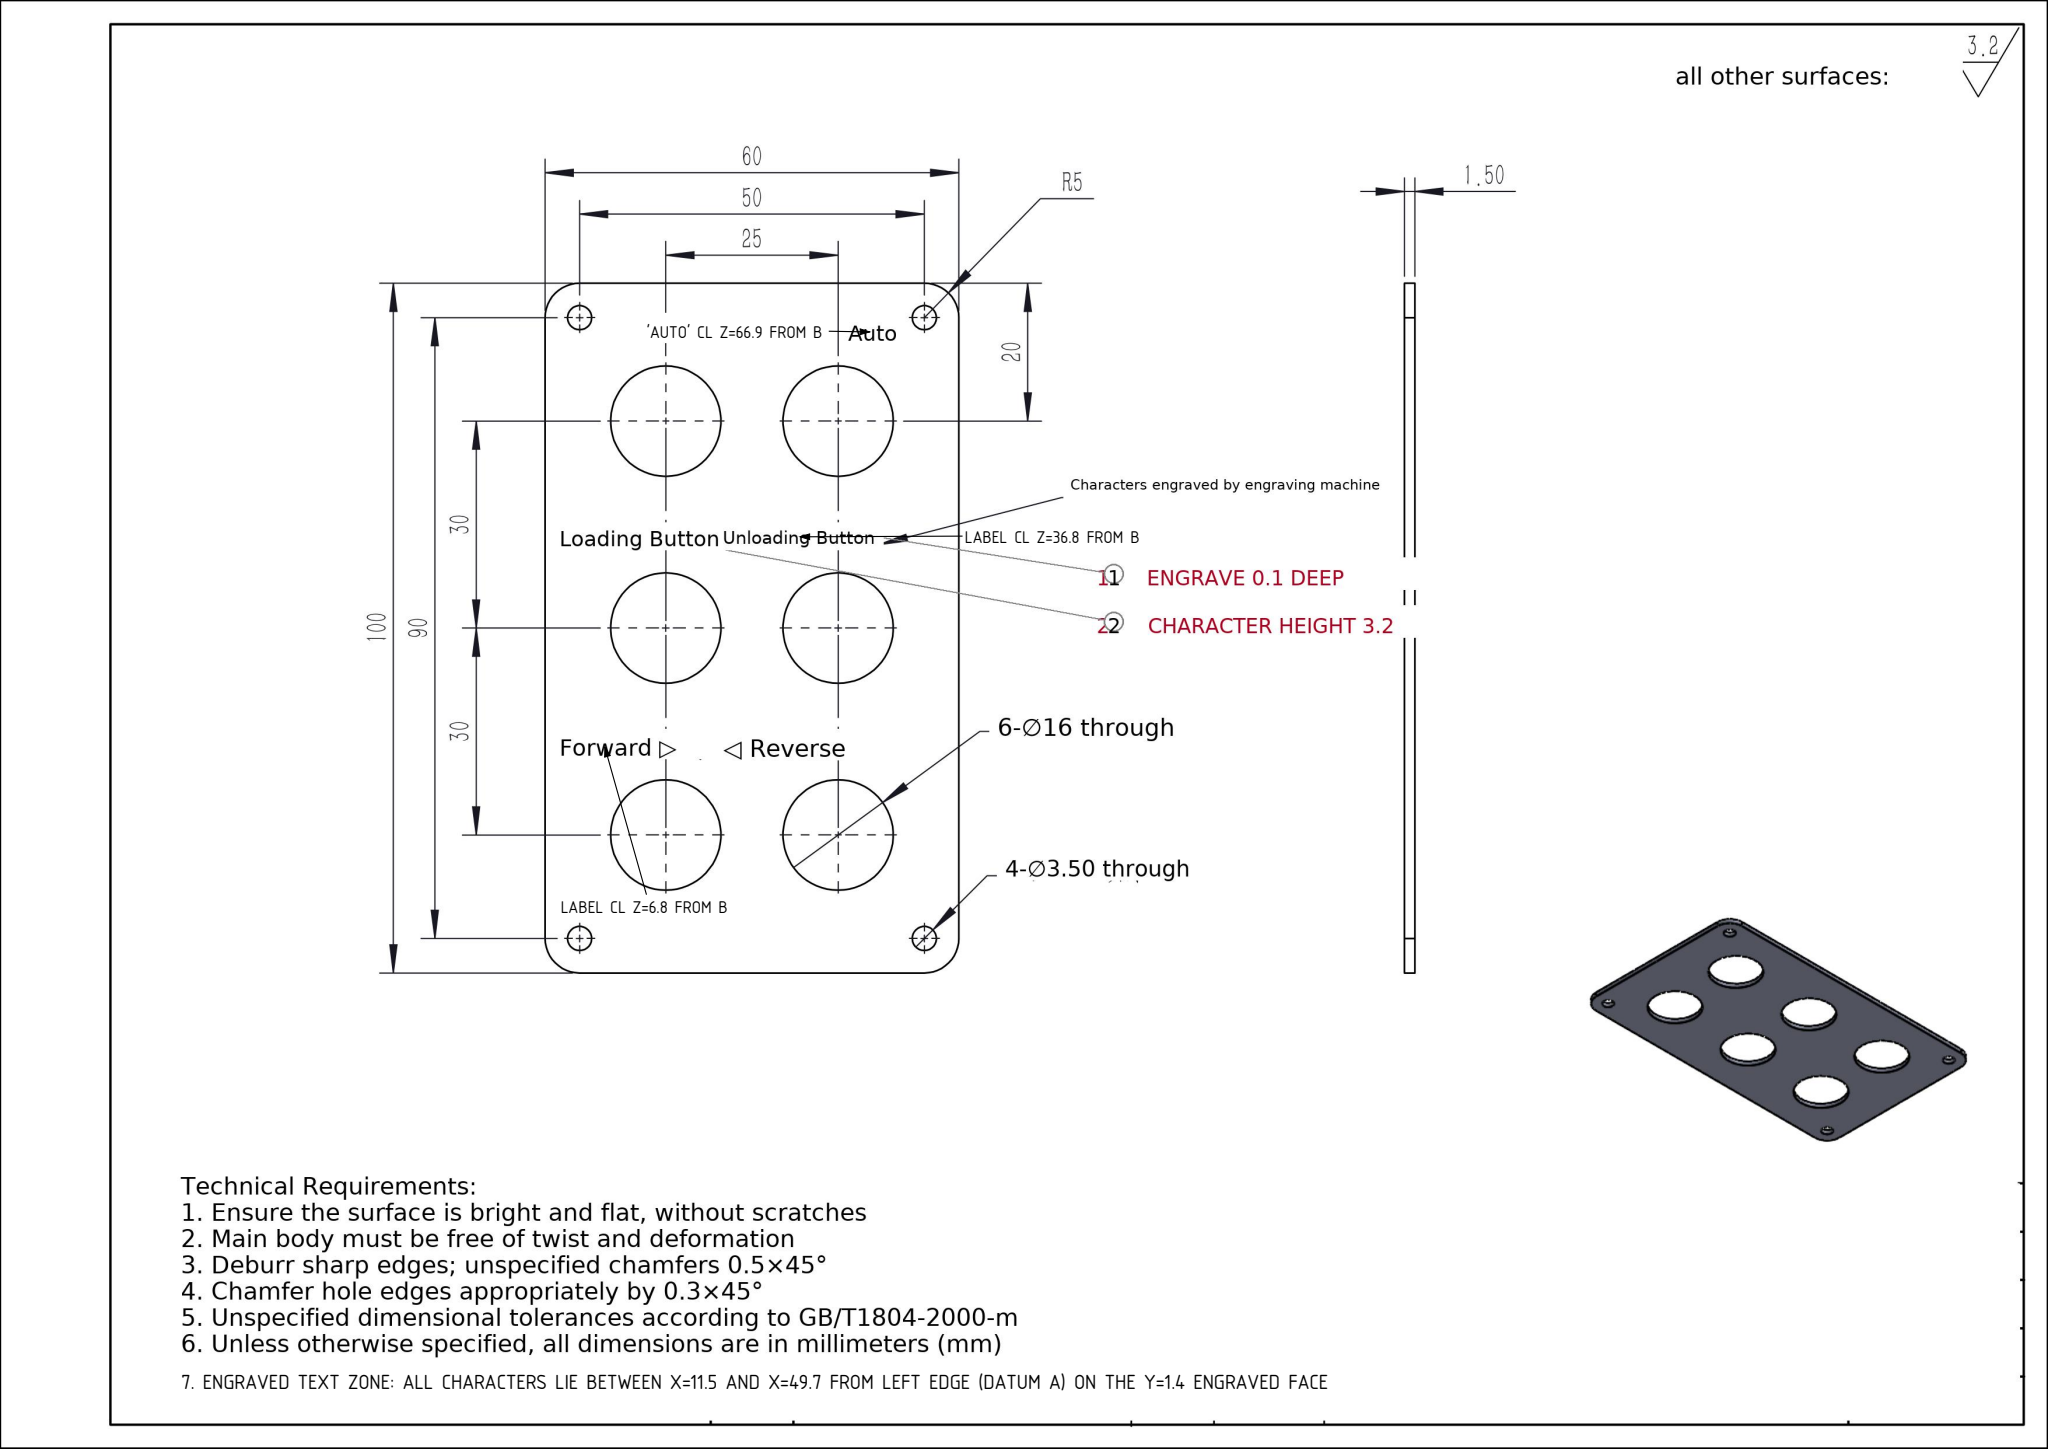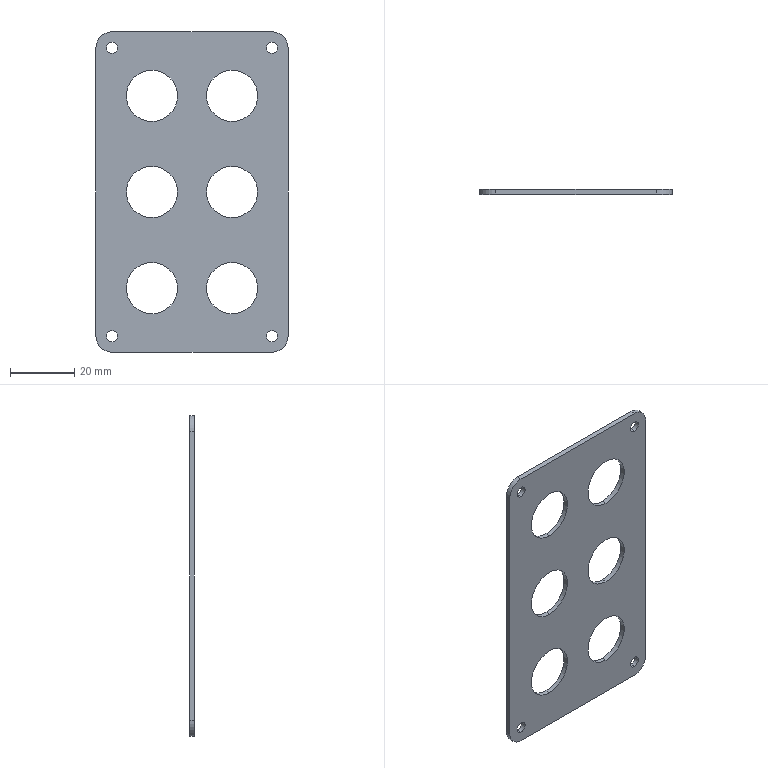Part | SolidWorks | mm | 1 solid | 1068 faces | box 60 x 1.5 x 100 mm | volume 7095 mm3 | plane 815 | spline 229 | cylinder 24 | commonest cylinder face diameters 16 x12 3.5 x8 10 x4
Drawing notes:
ENGRAVED TEXT ZONE: ALL CHARACTERS LIE BETWEEN X=11.5 AND X=49.7 FROM LEFT EDGE (DATUM A) ON THE Y=1.4 ENGRAVED FACE | from the solid: axis_planes normal x on engraved face range from 11.51 to 49.67
ENGRAVED LABEL 'AUTO': CHARACTER BAND Z=65.5 TO 68.2 FROM BOTTOM EDGE (DATUM B), CENTERLINE Z=66.9, i.e. 13.1 BELOW THE Ø16 HOLE AXIS AT Z=80; ENGRAVED FACE Y=1.4 | from the solid: axis_planes normal x at y[1.4,1.5] with z extents 65.5-68.2 (x 14.0-18.8); cylinders hole/bore Ø16 axis at (17.5/42.5, z=80)
ENGRAVED LABELS 'LOADING BUTTON'/'UNLOADING BUTTON': CHARACTER BAND Z=35.4 TO 38.1 FROM BOTTOM EDGE (DATUM B), CENTERLINE Z=36.8, i.e. 13.2 BELOW THE Ø16 HOLE AXES AT Z=50; ENGRAVED FACE Y=1.4 | from the solid: axis_planes normal x at y[1.4,1.5] with z extents 35.4-38.1 (x 12.1-48.2); cylinders hole/bore Ø16 axes at z=50
ENGRAVED LABELS 'FORWARD'/'REVERSE': CHARACTER BAND Z=5.4 TO 8.2 FROM BOTTOM EDGE (DATUM B), CENTERLINE Z=6.8, i.e. 13.2 BELOW THE Ø16 HOLE AXES AT Z=20; ENGRAVED FACE Y=1.4 | from the solid: axis_planes normal x at y[1.4,1.5] with z extents 5.4-8.2 (x 11.5-49.5); cylinders hole/bore Ø16 axes at z=20